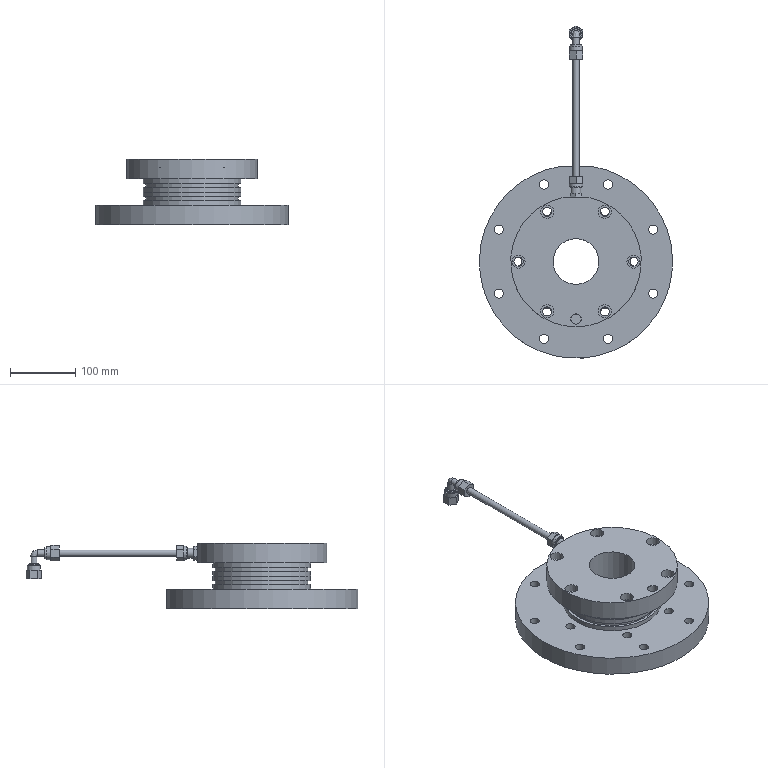Assembly | NX | mm | 5 component files | 5 solids | 207 faces | box 296 x 509 x 100 mm | volume 3082166 mm3 | plane 90 | cylinder 81 | cone 34 | spline 1 | torus 1 | commonest cylinder face diameters 20 x22 14 x20 10 x7 12 x6 150 x4 17 x3 6 x3 142 x2
Bill of materials:
CH3404.4-2 | 1 |  | Long, straight hollow cylindrical tube with a constant circular cross-section and a concentric through-bore.
CH3404.4-1 | 1 |  | Axisymmetric straight fitting-like body: a plain cylindrical tube stub, then a smaller hex section, a cylindrical neck with a stepped collar or groove, and a larger hex section at the opposite end, with a central through-bore.
CH3404.6-1 | 1 |  | Thick circular flange plate with a large central bore, a raised cylindrical boss on one face that has an external circumferential groove, and a pattern of axial through-holes.
CH3404.4-3 | 1 |  | 90-degree elbow fitting-like body: a bent tubular section joining two cylindrical/hexagonal end bodies, each with a hex section, collars, and an open bore.
CH3404.6-4 | 1 |  | Thick circular flange disc with a large central bore, seven axial through-holes on one circle, and a narrower cylindrical spigot on one face with an external circumferential groove.
Mates:
1. fix | CH3404_4-1 1 component
2. distance | CH3404_4-2 1 face | CH3404_4-1 1 face
3. touch align | CH3404_4-2 1 | assembly datumplane
4. touch align | CH3404_4-2 1 face | assembly datumaxis
5. distance | CH3404_4-3 1 face | CH3404_4-2 1 face
6. touch align | CH3404_4-3 1 | assembly datumplane
7. touch align | CH3404_4-3 1 face | assembly datumaxis
8. touch align | CH3404_6-1 1 face | CH3404_6-4 1 face